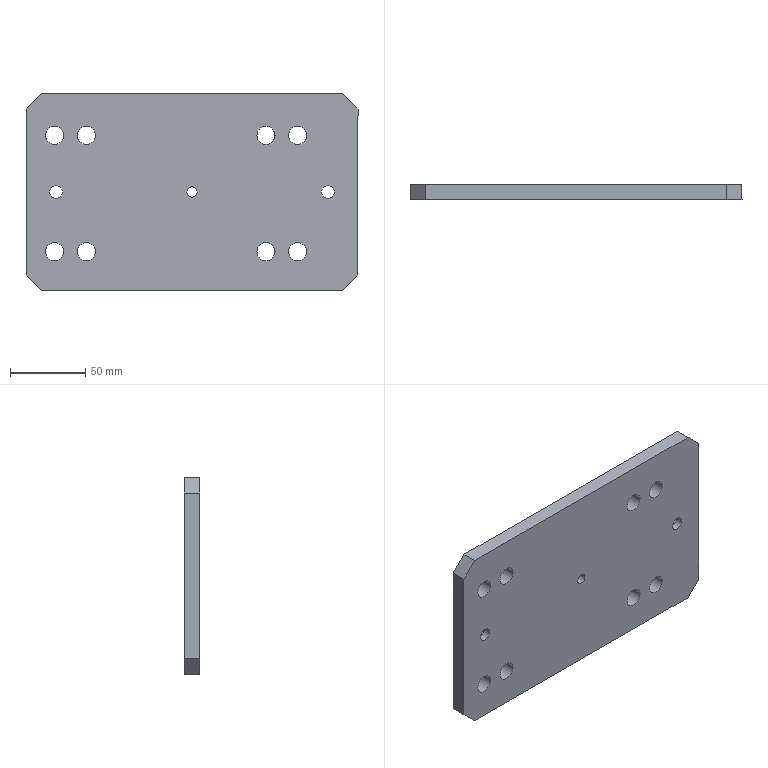Component | SolidWorks | AdsorptionRelease-1 | 1 solid | 38 faces | box 220 x 10.03 x 130 mm | volume 272011 mm3 | cylinder 26 | plane 12 | commonest cylinder face diameters 12 x16 8.5 x4 16 x4 6.8 x2
build123d program:
from build123d import *

# Parameters (mm, degrees)
SKETCH1_W                   = 220
SKETCH1_H                   = 130
BOSS_EXTRUDE1_DEPTH         = 10
M8_TAPPED_HOLE1_D           = 6.8
M8_TAPPED_HOLE1_DEPTH       = 19.75
M8_TAPPED_HOLE1_TIP         = 2.043
SKETCH4_R                   = 8
CUT_EXTRUDE1_DEPTH          = 5
SKETCH5_R                   = 4.25
CUT_EXTRUDE2_DEPTH          = 25
CHAMFER1_SIZE               = 10
M12X1_25_TAPPED_HOLE1_D     = 12
M12X1_25_TAPPED_HOLE1_DEPTH = 27.75
M12X1_25_TAPPED_HOLE1_TIP   = 3.605


with BuildPart() as part:
    # Sketch1 → Boss-Extrude1 (new body)
    with BuildSketch(Plane.XY):
        Rectangle(SKETCH1_W, SKETCH1_H)
    extrude(amount=BOSS_EXTRUDE1_DEPTH)

    # M8 Tapped Hole1
    with Locations(Plane.XY.offset(10)):
        with Locations((0, 0)):
            Hole(M8_TAPPED_HOLE1_D / 2, depth=M8_TAPPED_HOLE1_DEPTH)
            with Locations((0, 0, -(M8_TAPPED_HOLE1_DEPTH + M8_TAPPED_HOLE1_TIP / 2))):  # 118° drill point
                Cone(0, M8_TAPPED_HOLE1_D / 2, M8_TAPPED_HOLE1_TIP, mode=Mode.SUBTRACT)

    # Sketch4 → Cut-Extrude1 (cut)
    with BuildSketch(Plane.XY.offset(10)):
        with Locations((-90, 0)):
            Circle(SKETCH4_R)
        with Locations((90, 0)):
            Circle(SKETCH4_R)
    extrude(amount=-CUT_EXTRUDE1_DEPTH, mode=Mode.SUBTRACT)

    # Sketch5 → Cut-Extrude2 (cut)
    with BuildSketch(Plane(origin=(0, 0, 0), x_dir=(-1, 0, 0), z_dir=(0, 0, -1))):
        with Locations((-90, 0)):
            Circle(SKETCH5_R)
        with Locations((90, 0)):
            Circle(SKETCH5_R)
    extrude(amount=-CUT_EXTRUDE2_DEPTH, mode=Mode.SUBTRACT)

    # Chamfer1
    chamfer1_edges = [part.edges().sort_by_distance(p)[0] for p in [
        (-110, 65, 5),
        (110, 65, 5),
        (110, -65, 5),
        (-110, -65, 5),
    ]]
    chamfer(chamfer1_edges, length=CHAMFER1_SIZE)

    # M12x1.25 Tapped Hole1
    with Locations(Plane.XY.offset(10)):
        with Locations((70, 39.5), (49, 39.5), (-91, 39.5), (-70, 39.5), (49, -37.5), (70, -37.5), (-91, -37.5), (-70, -37.5)):
            Hole(M12X1_25_TAPPED_HOLE1_D / 2, depth=M12X1_25_TAPPED_HOLE1_DEPTH)
            with Locations((0, 0, -(M12X1_25_TAPPED_HOLE1_DEPTH + M12X1_25_TAPPED_HOLE1_TIP / 2))):  # 118° drill point
                Cone(0, M12X1_25_TAPPED_HOLE1_D / 2, M12X1_25_TAPPED_HOLE1_TIP, mode=Mode.SUBTRACT)


solid = part.part

# Placed as in the assembly
solid = solid.moved(Location((1702.148, 3931.47, 1079.241), (-90, -0.008895, 0)))